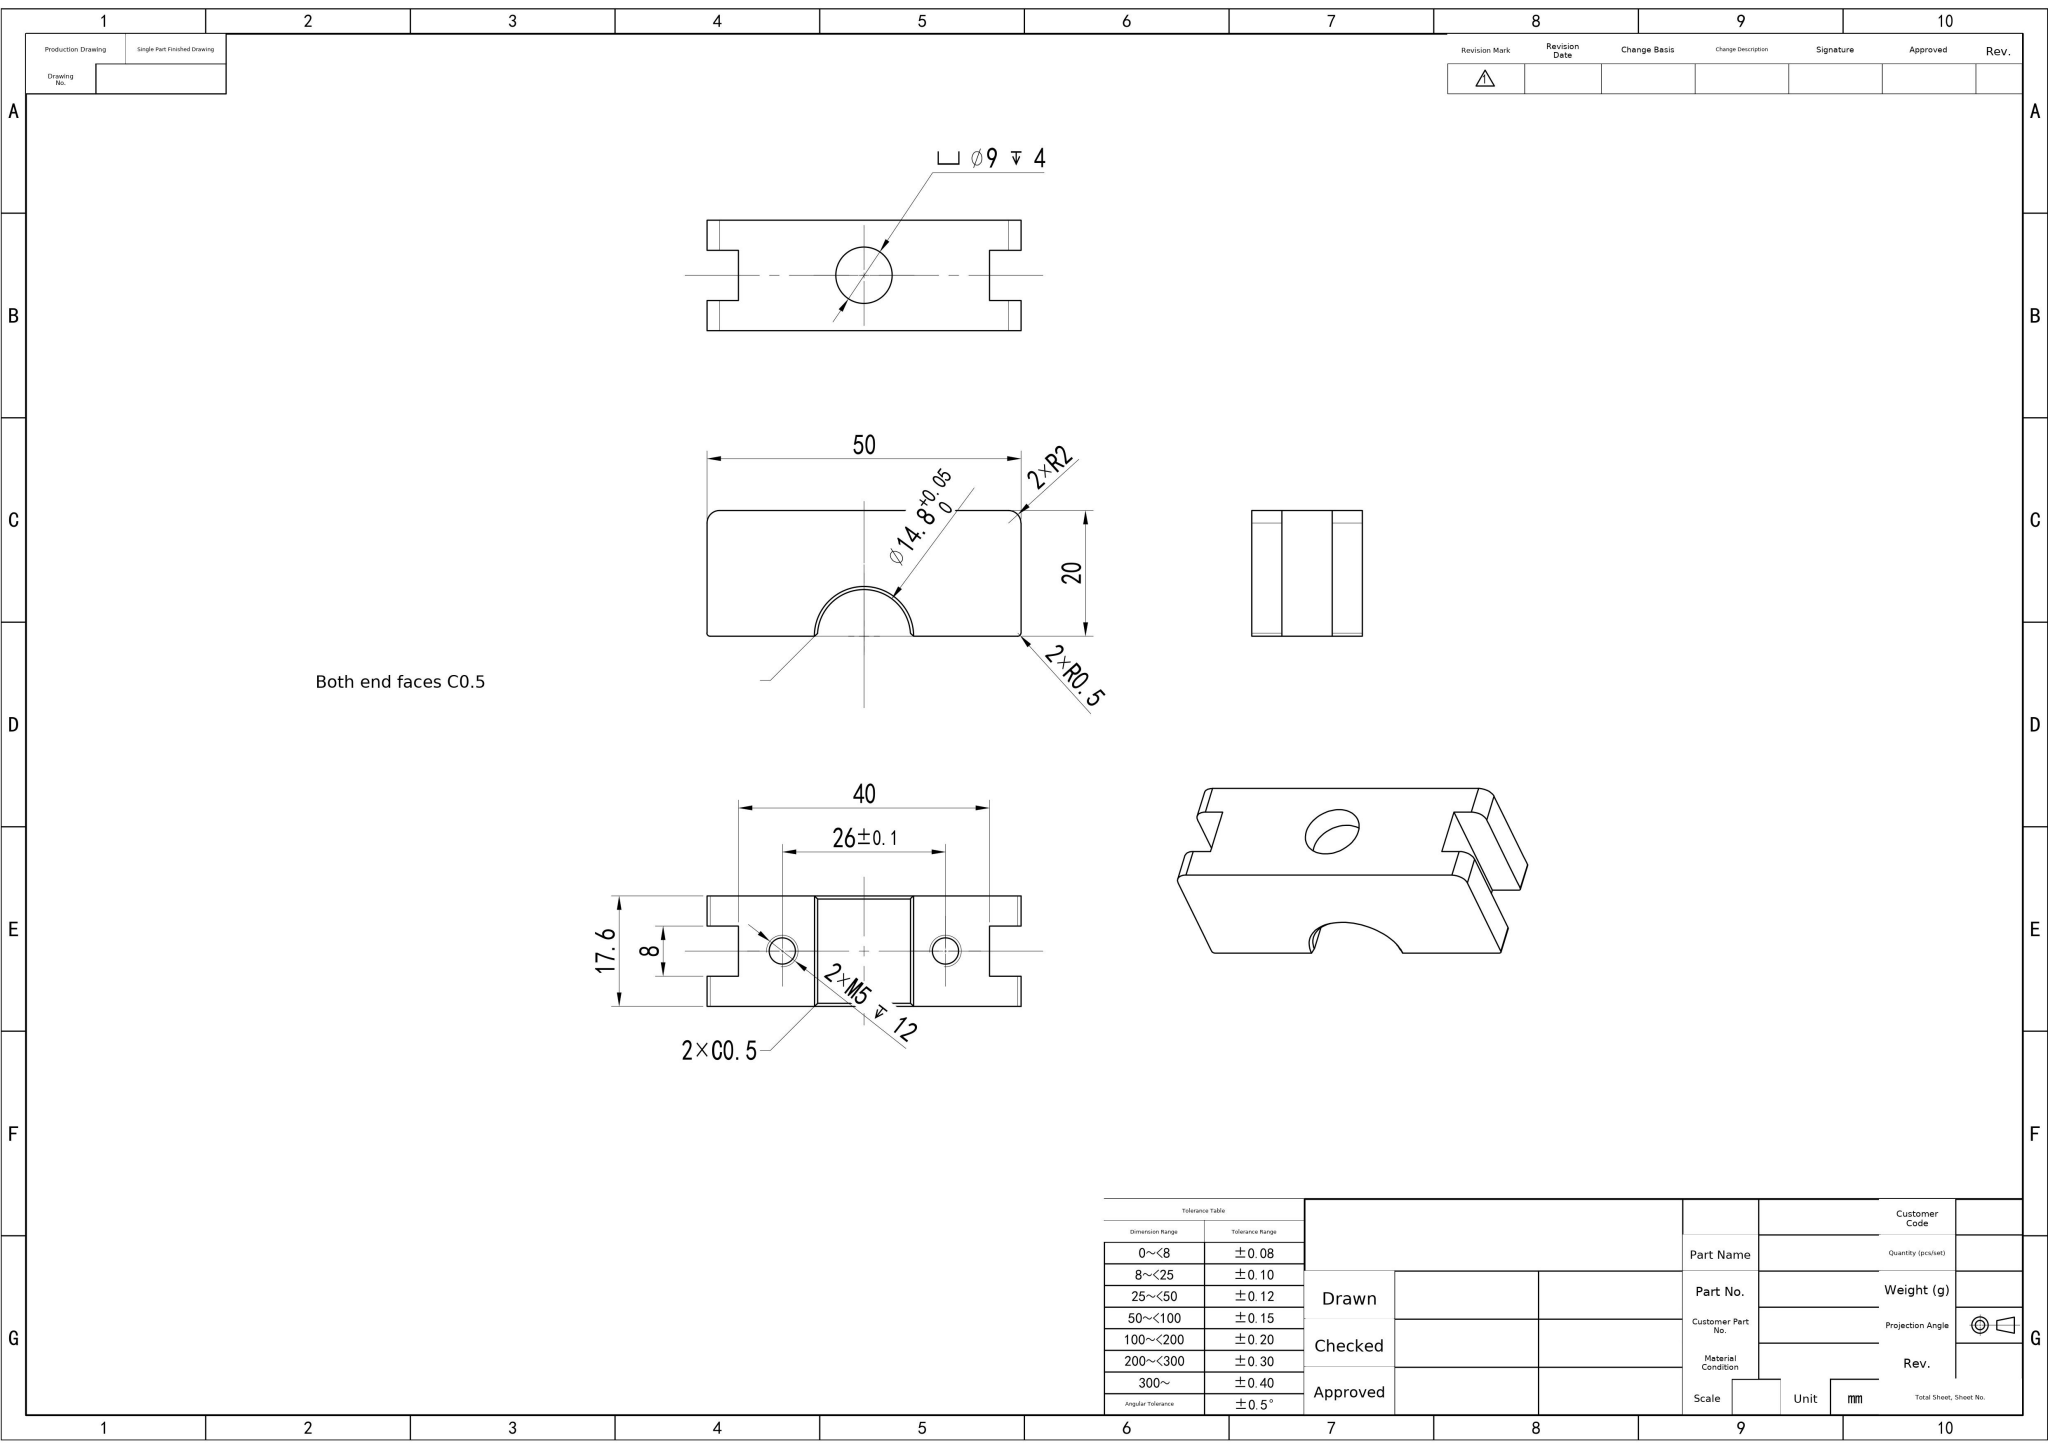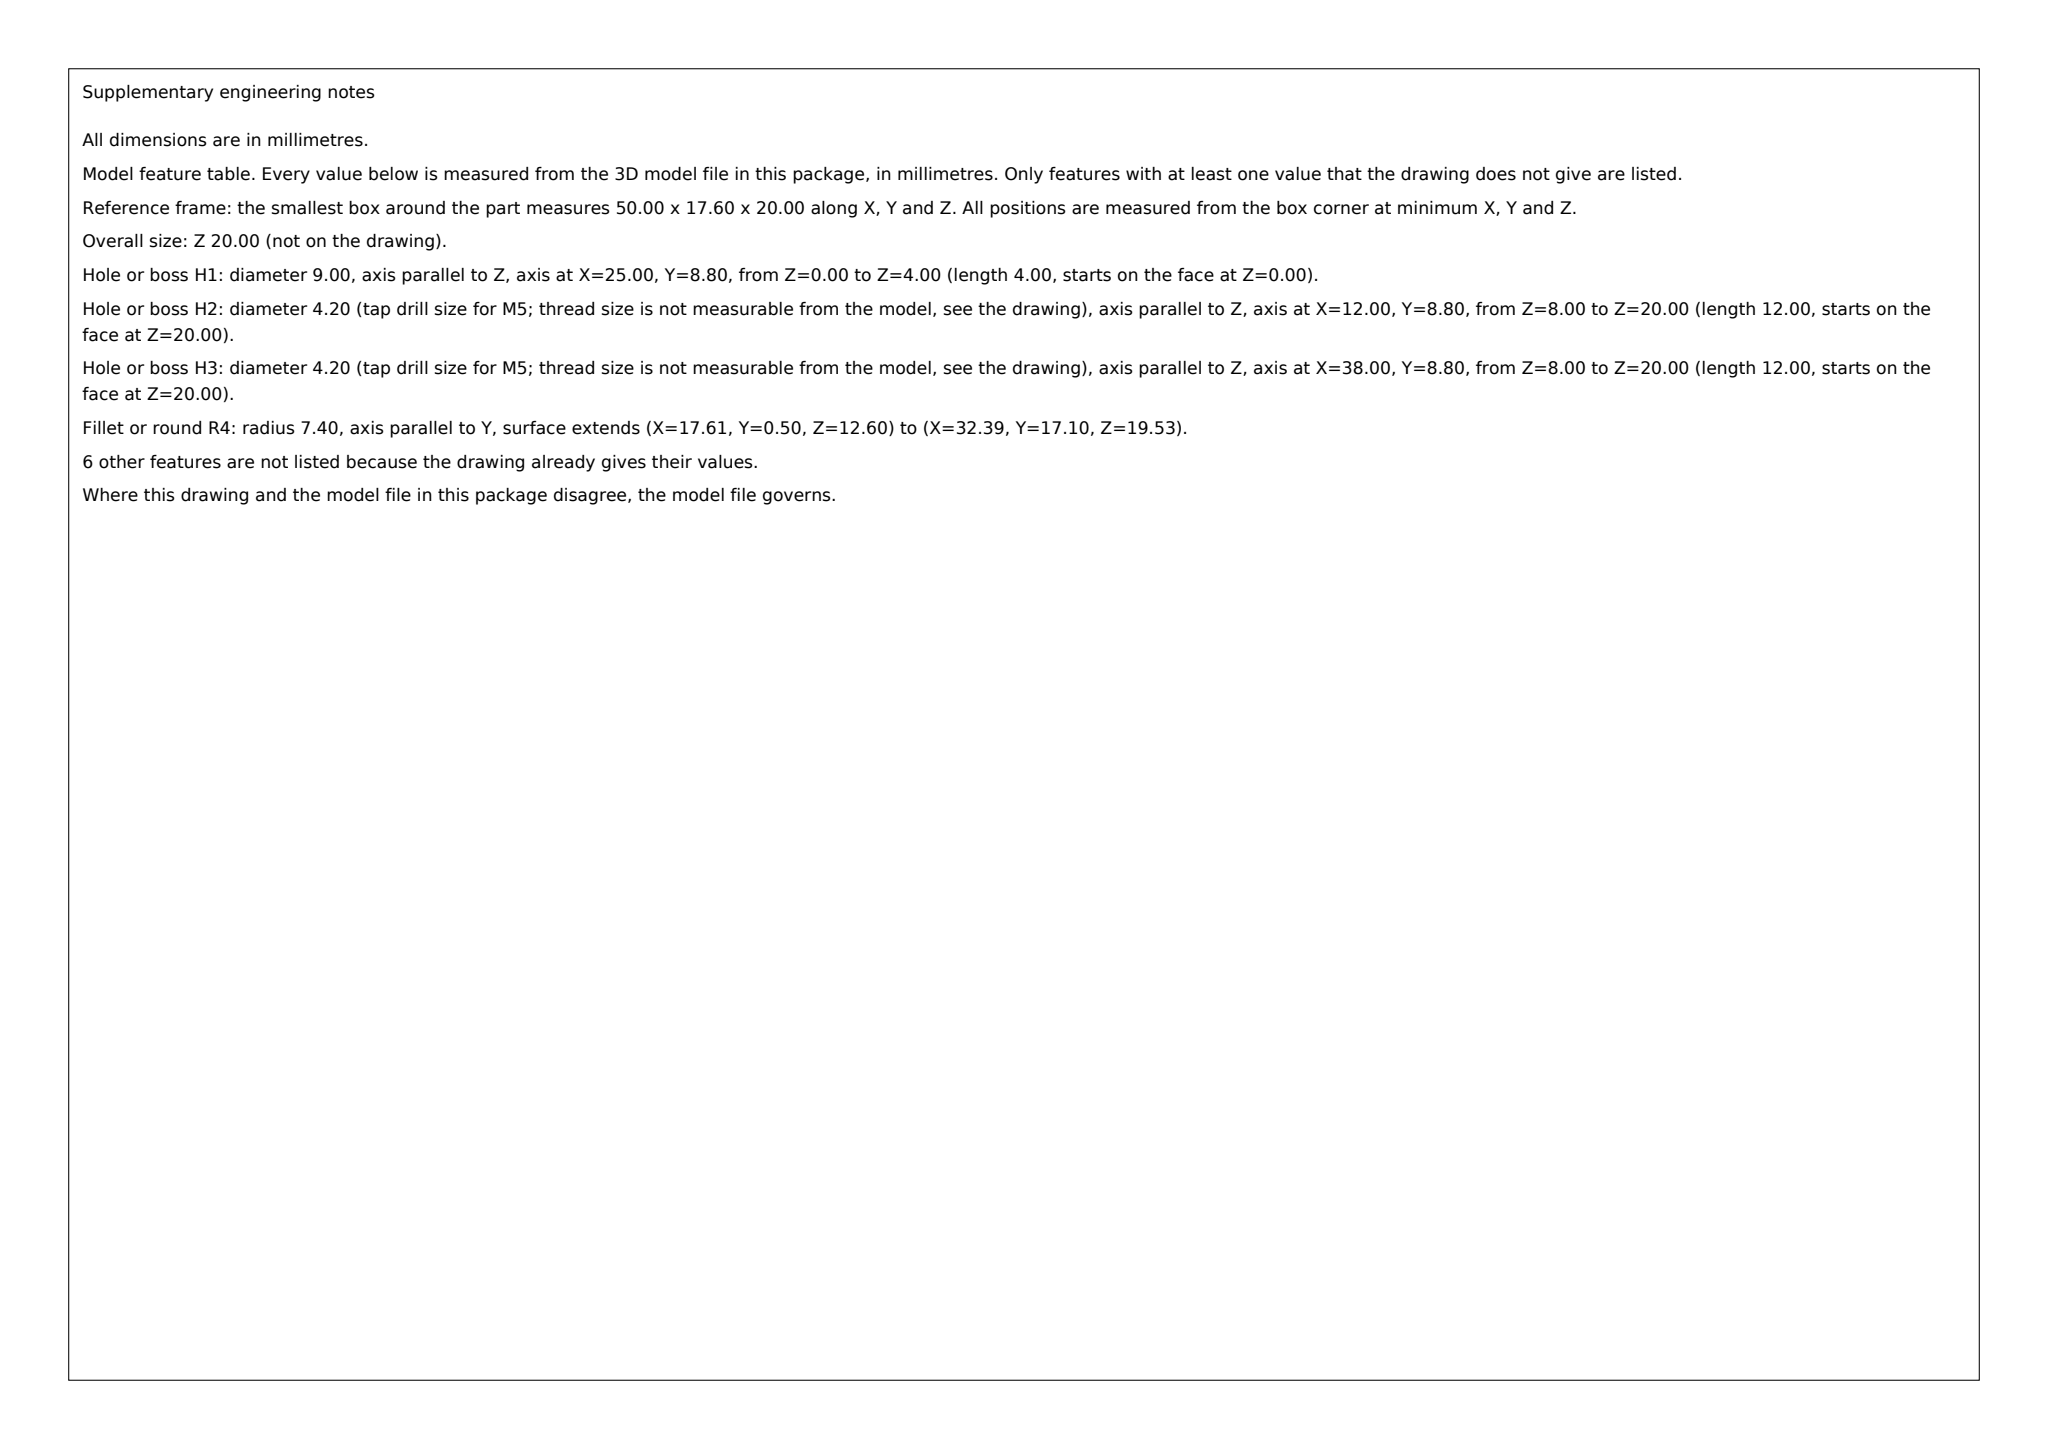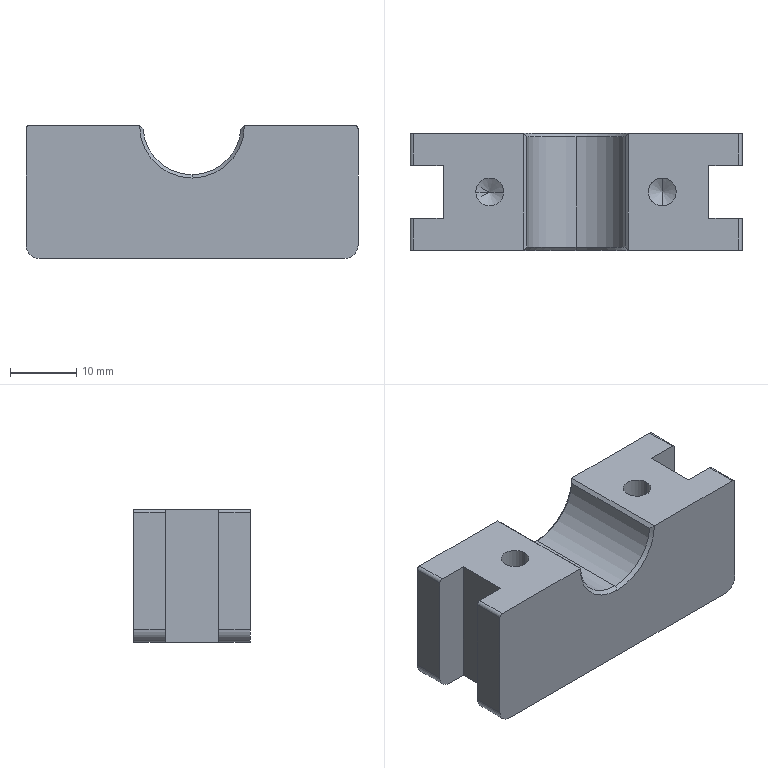Part | SolidWorks | mm | 1 solid | 41 faces | box 50 x 17.6 x 20 mm | volume 13860 mm3 | plane 18 | cylinder 16 | cone 7 | commonest cylinder face diameters 4.2 x4 4 x4 1 x4 9 x2 14.8 x2